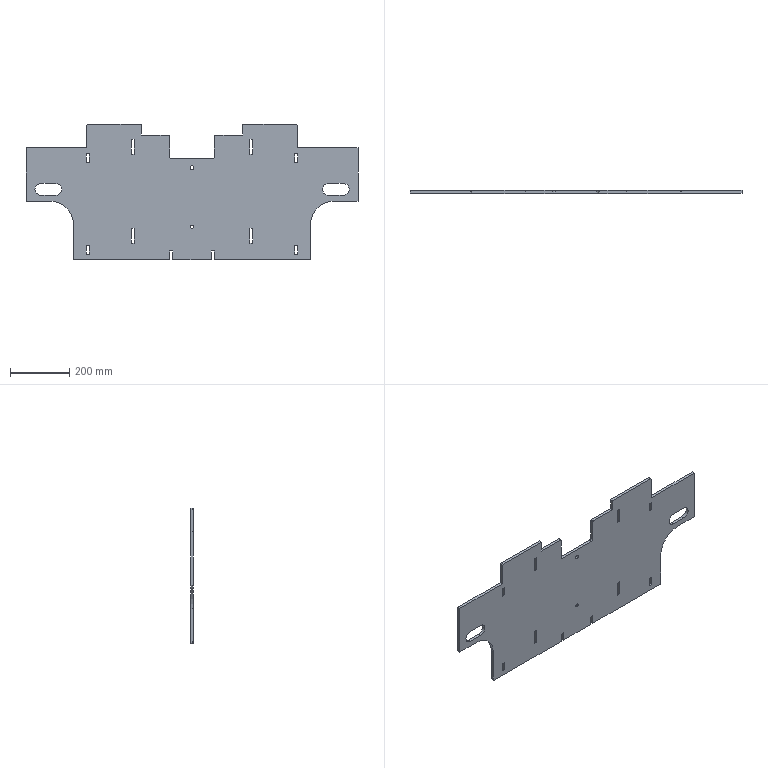Component | SolidWorks | LadderFixingPlate-1 | 1 solid | 92 faces | box 1120 x 10 x 458 mm | volume 3841821 mm3 | plane 74 | cylinder 18 | commonest cylinder face diameters 40 x6 10 x6 12.2 x2 10.6 x2 160 x2 | material Q235
build123d program:
from build123d import *

# Parameters (mm, degrees)
SKETCH1_2_R             = 5.3
SKETCH1_2_R_2           = 6.1
SKETCH1_2_W             = 10.2
SKETCH1_2_H             = 30
SKETCH1_2_W_2           = 10
SKETCH1_2_H_2           = 50
BOSS_EXTRUDE1_DEPTH     = 10
CUT_EXTRUDE1_DEPTH      = 762.48
CUT_EXTRUDE1_DEPTH_BACK = 762.48
SKETCH1_W               = 0.4
SKETCH1_H               = 1.6


with BuildPart() as part:
    # Sketch1_2 → Boss-Extrude1 (new body)
    with BuildSketch(Plane.XY):
        with BuildLine():
            Line((-237.296, -229.656), (-237.296, -234.656))
            Line((-237.296, -234.656), (-237.296, -236.192))
            ThreePointArc((-237.296, -236.192), (-235.832, -239.728), (-232.296, -241.192))
            Line((-232.296, -241.192), (87.204, -241.192))
            Line((87.204, -241.192), (87.204, -211.192))
            Line((87.204, -211.192), (97.204, -211.192))
            Line((97.204, -211.192), (97.704, -211.192))
            Line((97.704, -211.192), (97.704, -241.192))
            Line((97.704, -241.192), (226.704, -241.192))
            Line((226.704, -241.192), (226.704, -211.192))
            Line((226.704, -211.192), (227.204, -211.192))
            Line((227.204, -211.192), (237.204, -211.192))
            Line((237.204, -211.192), (237.204, -241.192))
            Line((237.204, -241.192), (556.704, -241.192))
            ThreePointArc((556.704, -241.192), (560.239, -239.728), (561.704, -236.192))
            Line((561.704, -236.192), (561.704, -234.656))
            Line((561.704, -234.656), (561.704, -229.656))
            Line((561.704, -229.656), (561.704, -123.192))
            ThreePointArc((561.704, -123.192), (585.135, -66.624), (641.704, -43.192))
            Line((641.704, -43.192), (722.204, -43.192))
            Line((722.204, -43.192), (722.204, 136.808))
            Line((722.204, 136.808), (517.704, 136.808))
            Line((517.704, 136.808), (517.704, 166.808))
            Line((517.704, 166.808), (517.704, 213.808))
            Line((517.704, 213.808), (514.704, 216.808))
            Line((514.704, 216.808), (333.204, 216.808))
            Line((333.204, 216.808), (333.204, 179.808))
            Line((333.204, 179.808), (242.204, 179.808))
            ThreePointArc((242.204, 179.808), (238.668, 178.343), (237.204, 174.808))
            Line((237.204, 174.808), (237.204, 104.808))
            ThreePointArc((237.204, 104.808), (235.739, 101.272), (232.204, 99.808))
            Line((232.204, 99.808), (92.204, 99.808))
            ThreePointArc((92.204, 99.808), (88.668, 101.272), (87.204, 104.808))
            Line((87.204, 104.808), (87.204, 174.808))
            ThreePointArc((87.204, 174.808), (85.739, 178.343), (82.204, 179.808))
            Line((82.204, 179.808), (-8.796, 179.808))
            Line((-8.796, 179.808), (-8.796, 216.808))
            Line((-8.796, 216.808), (-190.296, 216.808))
            Line((-190.296, 216.808), (-193.296, 213.808))
            Line((-193.296, 213.808), (-193.296, 166.808))
            Line((-193.296, 166.808), (-193.296, 136.808))
            Line((-193.296, 136.808), (-397.796, 136.808))
            Line((-397.796, 136.808), (-397.796, -43.192))
            Line((-397.796, -43.192), (-317.296, -43.192))
            ThreePointArc((-317.296, -43.192), (-260.728, -66.624), (-237.296, -123.192))
            Line((-237.296, -123.192), (-237.296, -229.656))
        make_face()
        with Locations((162.204, -129.656)):
            Circle(SKETCH1_2_R, mode=Mode.SUBTRACT)
        with Locations((162.204, 70.344)):
            Circle(SKETCH1_2_R_2, mode=Mode.SUBTRACT)
        Polygon((-194.896, 86.808), (-184.696, 86.808), (-184.696, 106.808), (-184.696, 116.808), (-194.896, 116.808), align=None, mode=Mode.SUBTRACT)
        with Locations((-189.796, -207.192)):
            Rectangle(SKETCH1_2_W, SKETCH1_2_H, mode=Mode.SUBTRACT)
        with BuildLine():
            Line((-347.797, 16.728), (-297.797, 16.728))
            ThreePointArc((-297.797, 16.728), (-277.797, -3.272), (-297.797, -23.272))
            Line((-297.797, -23.272), (-347.797, -23.272))
            ThreePointArc((-347.797, -23.272), (-367.797, -3.272), (-347.797, 16.728))
        make_face(mode=Mode.SUBTRACT)
        with Locations((-37.301, -160.005)):
            Rectangle(SKETCH1_2_W_2, SKETCH1_2_H_2, mode=Mode.SUBTRACT)
        with Locations((-37.301, 139.995)):
            Rectangle(SKETCH1_2_W_2, SKETCH1_2_H_2, mode=Mode.SUBTRACT)
        with Locations((361.699, -160.005)):
            Rectangle(SKETCH1_2_W_2, SKETCH1_2_H_2, mode=Mode.SUBTRACT)
        with Locations((361.699, 139.995)):
            Rectangle(SKETCH1_2_W_2, SKETCH1_2_H_2, mode=Mode.SUBTRACT)
        Polygon((519.304, 86.808), (509.104, 86.808), (509.104, 106.808), (509.104, 116.808), (519.304, 116.808), align=None, mode=Mode.SUBTRACT)
        with Locations((514.204, -207.192)):
            Rectangle(SKETCH1_2_W, SKETCH1_2_H, mode=Mode.SUBTRACT)
        with BuildLine():
            Line((672.204, 16.728), (622.204, 16.728))
            ThreePointArc((622.204, 16.728), (602.204, -3.272), (622.204, -23.272))
            Line((622.204, -23.272), (672.204, -23.272))
            ThreePointArc((672.204, -23.272), (692.204, -3.272), (672.204, 16.728))
        make_face(mode=Mode.SUBTRACT)
    extrude(amount=BOSS_EXTRUDE1_DEPTH)

    # Sketch1 → Cut-Extrude1 (cut, two sides: drawn at the far end of the back side and taken through both)
    with BuildSketch(Plane.XY.offset(-CUT_EXTRUDE1_DEPTH_BACK)):
        with Locations((97.858, -241.098)):
            Rectangle(SKETCH1_W, SKETCH1_H)
        with Locations((226.558, -241.098)):
            Rectangle(SKETCH1_W, SKETCH1_H)
    extrude(amount=CUT_EXTRUDE1_DEPTH + CUT_EXTRUDE1_DEPTH_BACK, mode=Mode.SUBTRACT)


solid = part.part

# Placed as in the assembly
solid = solid.moved(Location((-979.858, -1073.526, 2598.898), (90, 0, 0)))